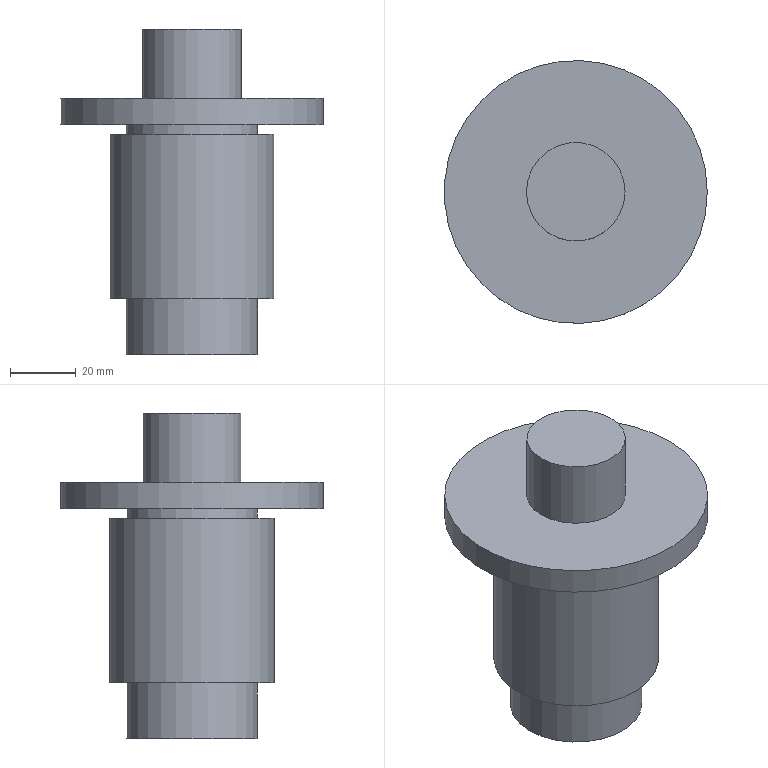Component | NX | SUPPORT_BASE | 1 solid | 11 faces | box 80 x 80 x 99 mm | volume 178364 mm3 | plane 6 | cylinder 5 | commonest cylinder face diameters 40 x2 50 x1 80 x1 30 x1
STEP:
#1=CARTESIAN_POINT('',(0.,0.,0.));
#2=DIRECTION('',(0.,0.,1.));
#3=DIRECTION('',(1.,0.,0.));
#4=AXIS2_PLACEMENT_3D('',#1,#2,#3);
#5=CARTESIAN_POINT('',(577.45,0.,4.));
#6=VERTEX_POINT('',#5);
#7=CARTESIAN_POINT('',(562.45,0.,4.));
#8=DIRECTION('',(0.,0.,1.));
#9=DIRECTION('',(1.,0.,0.));
#10=AXIS2_PLACEMENT_3D('',#7,#8,#9);
#11=CIRCLE('',#10,15.);
#12=CARTESIAN_POINT('',(562.45,0.,4.));
#13=DIRECTION('',(0.,0.,1.));
#14=DIRECTION('',(1.,0.,0.));
#15=AXIS2_PLACEMENT_3D('',#12,#13,#14);
#16=PLANE('',#15);
#17=CARTESIAN_POINT('',(0.,0.));
#18=DIRECTION('',(1.,0.));
#19=AXIS2_PLACEMENT_2D('',#17,#18);
#20=CIRCLE('',#19,15.);
#21=(GEOMETRIC_REPRESENTATION_CONTEXT(2)PARAMETRIC_REPRESENTATION_CONTEXT()REPRESENTATION_CONTEXT('',''));
#22=DEFINITIONAL_REPRESENTATION('',(#20),#21);
#23=PCURVE('',#16,#22);
#24=CARTESIAN_POINT('',(562.45,0.,4.));
#25=DIRECTION('',(0.,0.,1.));
#26=DIRECTION('',(1.,0.,0.));
#27=AXIS2_PLACEMENT_3D('',#24,#25,#26);
#28=CYLINDRICAL_SURFACE('',#27,15.);
#29=CARTESIAN_POINT('',(0.,0.));
#30=DIRECTION('',(1.,0.));
#31=VECTOR('',#30,1.);
#32=LINE('',#29,#31);
#33=(GEOMETRIC_REPRESENTATION_CONTEXT(2)PARAMETRIC_REPRESENTATION_CONTEXT()REPRESENTATION_CONTEXT('',''));
#34=DEFINITIONAL_REPRESENTATION('',(#32),#33);
#35=PCURVE('',#28,#34);
#36=SURFACE_CURVE('',#11,(#23,#35),.PCURVE_S1.);
#37=EDGE_CURVE('',#6,#6,#36,.T.);
#38=ORIENTED_EDGE('',*,*,#37,.T.);
#39=EDGE_LOOP('',(#38));
#40=FACE_BOUND('',#39,.T.);
#41=ADVANCED_FACE('',(#40),#16,.T.);
#42=CARTESIAN_POINT('',(582.45,0.,-95.));
#43=VERTEX_POINT('',#42);
#44=CARTESIAN_POINT('',(562.45,0.,-95.));
#45=DIRECTION('',(0.,0.,1.));
#46=DIRECTION('',(1.,0.,0.));
#47=AXIS2_PLACEMENT_3D('',#44,#45,#46);
#48=CIRCLE('',#47,20.);
#49=CARTESIAN_POINT('',(562.45,0.,-95.));
#50=DIRECTION('',(0.,0.,1.));
#51=DIRECTION('',(1.,0.,0.));
#52=AXIS2_PLACEMENT_3D('',#49,#50,#51);
#53=PLANE('',#52);
#54=CARTESIAN_POINT('',(0.,0.));
#55=DIRECTION('',(1.,0.));
#56=AXIS2_PLACEMENT_2D('',#54,#55);
#57=CIRCLE('',#56,20.);
#58=(GEOMETRIC_REPRESENTATION_CONTEXT(2)PARAMETRIC_REPRESENTATION_CONTEXT()REPRESENTATION_CONTEXT('',''));
#59=DEFINITIONAL_REPRESENTATION('',(#57),#58);
#60=PCURVE('',#53,#59);
#61=CARTESIAN_POINT('',(562.45,0.,4.));
#62=DIRECTION('',(0.,0.,1.));
#63=DIRECTION('',(1.,0.,0.));
#64=AXIS2_PLACEMENT_3D('',#61,#62,#63);
#65=CYLINDRICAL_SURFACE('',#64,20.);
#66=CARTESIAN_POINT('',(0.,-99.));
#67=DIRECTION('',(1.,0.));
#68=VECTOR('',#67,1.);
#69=LINE('',#66,#68);
#70=(GEOMETRIC_REPRESENTATION_CONTEXT(2)PARAMETRIC_REPRESENTATION_CONTEXT()REPRESENTATION_CONTEXT('',''));
#71=DEFINITIONAL_REPRESENTATION('',(#69),#70);
#72=PCURVE('',#65,#71);
#73=SURFACE_CURVE('',#48,(#60,#72),.PCURVE_S1.);
#74=EDGE_CURVE('',#43,#43,#73,.T.);
#75=ORIENTED_EDGE('',*,*,#74,.F.);
#76=EDGE_LOOP('',(#75));
#77=FACE_BOUND('',#76,.T.);
#78=ADVANCED_FACE('',(#77),#53,.F.);
#79=ORIENTED_EDGE('',*,*,#74,.T.);
#80=CARTESIAN_POINT('',(582.45,0.,-78.));
#81=VERTEX_POINT('',#80);
#82=CARTESIAN_POINT('',(582.45,0.,-95.));
#83=CARTESIAN_POINT('',(582.45,0.,-78.));
#84=B_SPLINE_CURVE_WITH_KNOTS('',1,(#82,#83),.UNSPECIFIED.,.F.,.F.,(2,2),(-99.,-82.),.PIECEWISE_BEZIER_KNOTS.);
#85=CARTESIAN_POINT('',(6.283,0.));
#86=DIRECTION('',(0.,1.));
#87=VECTOR('',#86,1.);
#88=LINE('',#85,#87);
#89=(GEOMETRIC_REPRESENTATION_CONTEXT(2)PARAMETRIC_REPRESENTATION_CONTEXT()REPRESENTATION_CONTEXT('',''));
#90=DEFINITIONAL_REPRESENTATION('',(#88),#89);
#91=PCURVE('',#65,#90);
#92=CARTESIAN_POINT('',(0.,0.));
#93=DIRECTION('',(0.,1.));
#94=VECTOR('',#93,1.);
#95=LINE('',#92,#94);
#96=(GEOMETRIC_REPRESENTATION_CONTEXT(2)PARAMETRIC_REPRESENTATION_CONTEXT()REPRESENTATION_CONTEXT('',''));
#97=DEFINITIONAL_REPRESENTATION('',(#95),#96);
#98=PCURVE('',#65,#97);
#99=SEAM_CURVE('',#84,(#91,#98),.PCURVE_S1.);
#100=EDGE_CURVE('',#43,#81,#99,.T.);
#101=ORIENTED_EDGE('',*,*,#100,.T.);
#102=CARTESIAN_POINT('',(562.45,0.,-78.));
#103=DIRECTION('',(0.,0.,1.));
#104=DIRECTION('',(1.,0.,0.));
#105=AXIS2_PLACEMENT_3D('',#102,#103,#104);
#106=CIRCLE('',#105,20.);
#107=CARTESIAN_POINT('',(0.,-82.));
#108=DIRECTION('',(1.,0.));
#109=VECTOR('',#108,1.);
#110=LINE('',#107,#109);
#111=(GEOMETRIC_REPRESENTATION_CONTEXT(2)PARAMETRIC_REPRESENTATION_CONTEXT()REPRESENTATION_CONTEXT('',''));
#112=DEFINITIONAL_REPRESENTATION('',(#110),#111);
#113=PCURVE('',#65,#112);
#114=CARTESIAN_POINT('',(562.45,-25.,-78.));
#115=DIRECTION('',(0.,0.,-1.));
#116=DIRECTION('',(-1.,0.,0.));
#117=AXIS2_PLACEMENT_3D('',#114,#115,#116);
#118=PLANE('',#117);
#119=CARTESIAN_POINT('',(-20.,25.));
#120=CARTESIAN_POINT('',(-20.,59.641));
#121=CARTESIAN_POINT('',(10.,42.321));
#122=CARTESIAN_POINT('',(40.,25.));
#123=CARTESIAN_POINT('',(10.,7.679));
#124=CARTESIAN_POINT('',(-20.,-9.641));
#125=CARTESIAN_POINT('',(-20.,25.));
#126=(BOUNDED_CURVE()B_SPLINE_CURVE(2,(#119,#120,#121,#122,#123,#124,#125),.UNSPECIFIED.,.T.,.F.)B_SPLINE_CURVE_WITH_KNOTS((1,2,2,2,2,1),(-2.094,0.,2.094,4.189,6.283,8.378),.UNSPECIFIED.)CURVE()GEOMETRIC_REPRESENTATION_ITEM()RATIONAL_B_SPLINE_CURVE((1.,0.5,1.,0.5,1.,0.5,1.))REPRESENTATION_ITEM(''));
#127=(GEOMETRIC_REPRESENTATION_CONTEXT(2)PARAMETRIC_REPRESENTATION_CONTEXT()REPRESENTATION_CONTEXT('',''));
#128=DEFINITIONAL_REPRESENTATION('',(#126),#127);
#129=PCURVE('',#118,#128);
#130=SURFACE_CURVE('',#106,(#113,#129),.PCURVE_S1.);
#131=EDGE_CURVE('',#81,#81,#130,.T.);
#132=ORIENTED_EDGE('',*,*,#131,.F.);
#133=ORIENTED_EDGE('',*,*,#100,.F.);
#134=EDGE_LOOP('',(#79,#101,#132,#133));
#135=FACE_BOUND('',#134,.T.);
#136=ADVANCED_FACE('',(#135),#65,.T.);
#137=ORIENTED_EDGE('',*,*,#131,.T.);
#138=EDGE_LOOP('',(#137));
#139=FACE_BOUND('',#138,.T.);
#140=CARTESIAN_POINT('',(587.45,0.,-78.));
#141=VERTEX_POINT('',#140);
#142=CARTESIAN_POINT('',(562.45,0.,-78.));
#143=DIRECTION('',(0.,0.,1.));
#144=DIRECTION('',(1.,0.,0.));
#145=AXIS2_PLACEMENT_3D('',#142,#143,#144);
#146=CIRCLE('',#145,25.);
#147=CARTESIAN_POINT('',(-25.,25.));
#148=CARTESIAN_POINT('',(-25.,68.301));
#149=CARTESIAN_POINT('',(12.5,46.651));
#150=CARTESIAN_POINT('',(50.,25.));
#151=CARTESIAN_POINT('',(12.5,3.349));
#152=CARTESIAN_POINT('',(-25.,-18.301));
#153=CARTESIAN_POINT('',(-25.,25.));
#154=(BOUNDED_CURVE()B_SPLINE_CURVE(2,(#147,#148,#149,#150,#151,#152,#153),.UNSPECIFIED.,.T.,.F.)B_SPLINE_CURVE_WITH_KNOTS((1,2,2,2,2,1),(-2.094,0.,2.094,4.189,6.283,8.378),.UNSPECIFIED.)CURVE()GEOMETRIC_REPRESENTATION_ITEM()RATIONAL_B_SPLINE_CURVE((1.,0.5,1.,0.5,1.,0.5,1.))REPRESENTATION_ITEM(''));
#155=(GEOMETRIC_REPRESENTATION_CONTEXT(2)PARAMETRIC_REPRESENTATION_CONTEXT()REPRESENTATION_CONTEXT('',''));
#156=DEFINITIONAL_REPRESENTATION('',(#154),#155);
#157=PCURVE('',#118,#156);
#158=CARTESIAN_POINT('',(562.45,0.,4.));
#159=DIRECTION('',(0.,0.,1.));
#160=DIRECTION('',(1.,0.,0.));
#161=AXIS2_PLACEMENT_3D('',#158,#159,#160);
#162=CYLINDRICAL_SURFACE('',#161,25.);
#163=CARTESIAN_POINT('',(0.,-82.));
#164=DIRECTION('',(1.,0.));
#165=VECTOR('',#164,1.);
#166=LINE('',#163,#165);
#167=(GEOMETRIC_REPRESENTATION_CONTEXT(2)PARAMETRIC_REPRESENTATION_CONTEXT()REPRESENTATION_CONTEXT('',''));
#168=DEFINITIONAL_REPRESENTATION('',(#166),#167);
#169=PCURVE('',#162,#168);
#170=SURFACE_CURVE('',#146,(#157,#169),.PCURVE_S1.);
#171=EDGE_CURVE('',#141,#141,#170,.T.);
#172=ORIENTED_EDGE('',*,*,#171,.F.);
#173=EDGE_LOOP('',(#172));
#174=FACE_BOUND('',#173,.T.);
#175=ADVANCED_FACE('',(#139,#174),#118,.T.);
#176=ORIENTED_EDGE('',*,*,#171,.T.);
#177=CARTESIAN_POINT('',(587.45,0.,-28.));
#178=VERTEX_POINT('',#177);
#179=CARTESIAN_POINT('',(587.45,0.,-78.));
#180=CARTESIAN_POINT('',(587.45,0.,-28.));
#181=B_SPLINE_CURVE_WITH_KNOTS('',1,(#179,#180),.UNSPECIFIED.,.F.,.F.,(2,2),(-82.,-32.),.PIECEWISE_BEZIER_KNOTS.);
#182=CARTESIAN_POINT('',(6.283,0.));
#183=DIRECTION('',(0.,1.));
#184=VECTOR('',#183,1.);
#185=LINE('',#182,#184);
#186=(GEOMETRIC_REPRESENTATION_CONTEXT(2)PARAMETRIC_REPRESENTATION_CONTEXT()REPRESENTATION_CONTEXT('',''));
#187=DEFINITIONAL_REPRESENTATION('',(#185),#186);
#188=PCURVE('',#162,#187);
#189=CARTESIAN_POINT('',(0.,0.));
#190=DIRECTION('',(0.,1.));
#191=VECTOR('',#190,1.);
#192=LINE('',#189,#191);
#193=(GEOMETRIC_REPRESENTATION_CONTEXT(2)PARAMETRIC_REPRESENTATION_CONTEXT()REPRESENTATION_CONTEXT('',''));
#194=DEFINITIONAL_REPRESENTATION('',(#192),#193);
#195=PCURVE('',#162,#194);
#196=SEAM_CURVE('',#181,(#188,#195),.PCURVE_S1.);
#197=EDGE_CURVE('',#141,#178,#196,.T.);
#198=ORIENTED_EDGE('',*,*,#197,.T.);
#199=CARTESIAN_POINT('',(562.45,0.,-28.));
#200=DIRECTION('',(0.,0.,1.));
#201=DIRECTION('',(1.,0.,0.));
#202=AXIS2_PLACEMENT_3D('',#199,#200,#201);
#203=CIRCLE('',#202,25.);
#204=CARTESIAN_POINT('',(0.,-32.));
#205=DIRECTION('',(1.,0.));
#206=VECTOR('',#205,1.);
#207=LINE('',#204,#206);
#208=(GEOMETRIC_REPRESENTATION_CONTEXT(2)PARAMETRIC_REPRESENTATION_CONTEXT()REPRESENTATION_CONTEXT('',''));
#209=DEFINITIONAL_REPRESENTATION('',(#207),#208);
#210=PCURVE('',#162,#209);
#211=CARTESIAN_POINT('',(562.45,-20.,-28.));
#212=DIRECTION('',(0.,0.,1.));
#213=DIRECTION('',(1.,0.,0.));
#214=AXIS2_PLACEMENT_3D('',#211,#212,#213);
#215=PLANE('',#214);
#216=CARTESIAN_POINT('',(0.,20.));
#217=DIRECTION('',(1.,0.));
#218=AXIS2_PLACEMENT_2D('',#216,#217);
#219=CIRCLE('',#218,25.);
#220=(GEOMETRIC_REPRESENTATION_CONTEXT(2)PARAMETRIC_REPRESENTATION_CONTEXT()REPRESENTATION_CONTEXT('',''));
#221=DEFINITIONAL_REPRESENTATION('',(#219),#220);
#222=PCURVE('',#215,#221);
#223=SURFACE_CURVE('',#203,(#210,#222),.PCURVE_S1.);
#224=EDGE_CURVE('',#178,#178,#223,.T.);
#225=ORIENTED_EDGE('',*,*,#224,.F.);
#226=ORIENTED_EDGE('',*,*,#197,.F.);
#227=EDGE_LOOP('',(#176,#198,#225,#226));
#228=FACE_BOUND('',#227,.T.);
#229=ADVANCED_FACE('',(#228),#162,.T.);
#230=ORIENTED_EDGE('',*,*,#224,.T.);
#231=EDGE_LOOP('',(#230));
#232=FACE_BOUND('',#231,.T.);
#233=CARTESIAN_POINT('',(582.45,0.,-28.));
#234=VERTEX_POINT('',#233);
#235=CARTESIAN_POINT('',(562.45,0.,-28.));
#236=DIRECTION('',(0.,0.,1.));
#237=DIRECTION('',(1.,0.,0.));
#238=AXIS2_PLACEMENT_3D('',#235,#236,#237);
#239=CIRCLE('',#238,20.);
#240=CARTESIAN_POINT('',(0.,20.));
#241=DIRECTION('',(1.,0.));
#242=AXIS2_PLACEMENT_2D('',#240,#241);
#243=CIRCLE('',#242,20.);
#244=(GEOMETRIC_REPRESENTATION_CONTEXT(2)PARAMETRIC_REPRESENTATION_CONTEXT()REPRESENTATION_CONTEXT('',''));
#245=DEFINITIONAL_REPRESENTATION('',(#243),#244);
#246=PCURVE('',#215,#245);
#247=CARTESIAN_POINT('',(562.45,0.,4.));
#248=DIRECTION('',(0.,0.,1.));
#249=DIRECTION('',(1.,0.,0.));
#250=AXIS2_PLACEMENT_3D('',#247,#248,#249);
#251=CYLINDRICAL_SURFACE('',#250,20.);
#252=CARTESIAN_POINT('',(0.,-32.));
#253=DIRECTION('',(1.,0.));
#254=VECTOR('',#253,1.);
#255=LINE('',#252,#254);
#256=(GEOMETRIC_REPRESENTATION_CONTEXT(2)PARAMETRIC_REPRESENTATION_CONTEXT()REPRESENTATION_CONTEXT('',''));
#257=DEFINITIONAL_REPRESENTATION('',(#255),#256);
#258=PCURVE('',#251,#257);
#259=SURFACE_CURVE('',#239,(#246,#258),.PCURVE_S1.);
#260=EDGE_CURVE('',#234,#234,#259,.T.);
#261=ORIENTED_EDGE('',*,*,#260,.F.);
#262=EDGE_LOOP('',(#261));
#263=FACE_BOUND('',#262,.T.);
#264=ADVANCED_FACE('',(#232,#263),#215,.T.);
#265=ORIENTED_EDGE('',*,*,#260,.T.);
#266=CARTESIAN_POINT('',(582.45,0.,-25.));
#267=VERTEX_POINT('',#266);
#268=CARTESIAN_POINT('',(582.45,0.,-28.));
#269=CARTESIAN_POINT('',(582.45,0.,-25.));
#270=B_SPLINE_CURVE_WITH_KNOTS('',1,(#268,#269),.UNSPECIFIED.,.F.,.F.,(2,2),(-32.,-29.),.PIECEWISE_BEZIER_KNOTS.);
#271=CARTESIAN_POINT('',(6.283,0.));
#272=DIRECTION('',(0.,1.));
#273=VECTOR('',#272,1.);
#274=LINE('',#271,#273);
#275=(GEOMETRIC_REPRESENTATION_CONTEXT(2)PARAMETRIC_REPRESENTATION_CONTEXT()REPRESENTATION_CONTEXT('',''));
#276=DEFINITIONAL_REPRESENTATION('',(#274),#275);
#277=PCURVE('',#251,#276);
#278=CARTESIAN_POINT('',(0.,0.));
#279=DIRECTION('',(0.,1.));
#280=VECTOR('',#279,1.);
#281=LINE('',#278,#280);
#282=(GEOMETRIC_REPRESENTATION_CONTEXT(2)PARAMETRIC_REPRESENTATION_CONTEXT()REPRESENTATION_CONTEXT('',''));
#283=DEFINITIONAL_REPRESENTATION('',(#281),#282);
#284=PCURVE('',#251,#283);
#285=SEAM_CURVE('',#270,(#277,#284),.PCURVE_S1.);
#286=EDGE_CURVE('',#234,#267,#285,.T.);
#287=ORIENTED_EDGE('',*,*,#286,.T.);
#288=CARTESIAN_POINT('',(562.45,0.,-25.));
#289=DIRECTION('',(0.,0.,1.));
#290=DIRECTION('',(1.,0.,0.));
#291=AXIS2_PLACEMENT_3D('',#288,#289,#290);
#292=CIRCLE('',#291,20.);
#293=CARTESIAN_POINT('',(0.,-29.));
#294=DIRECTION('',(1.,0.));
#295=VECTOR('',#294,1.);
#296=LINE('',#293,#295);
#297=(GEOMETRIC_REPRESENTATION_CONTEXT(2)PARAMETRIC_REPRESENTATION_CONTEXT()REPRESENTATION_CONTEXT('',''));
#298=DEFINITIONAL_REPRESENTATION('',(#296),#297);
#299=PCURVE('',#251,#298);
#300=CARTESIAN_POINT('',(562.45,-40.,-25.));
#301=DIRECTION('',(0.,0.,-1.));
#302=DIRECTION('',(-1.,0.,0.));
#303=AXIS2_PLACEMENT_3D('',#300,#301,#302);
#304=PLANE('',#303);
#305=CARTESIAN_POINT('',(-20.,40.));
#306=CARTESIAN_POINT('',(-20.,74.641));
#307=CARTESIAN_POINT('',(10.,57.321));
#308=CARTESIAN_POINT('',(40.,40.));
#309=CARTESIAN_POINT('',(10.,22.679));
#310=CARTESIAN_POINT('',(-20.,5.359));
#311=CARTESIAN_POINT('',(-20.,40.));
#312=(BOUNDED_CURVE()B_SPLINE_CURVE(2,(#305,#306,#307,#308,#309,#310,#311),.UNSPECIFIED.,.T.,.F.)B_SPLINE_CURVE_WITH_KNOTS((1,2,2,2,2,1),(-2.094,0.,2.094,4.189,6.283,8.378),.UNSPECIFIED.)CURVE()GEOMETRIC_REPRESENTATION_ITEM()RATIONAL_B_SPLINE_CURVE((1.,0.5,1.,0.5,1.,0.5,1.))REPRESENTATION_ITEM(''));
#313=(GEOMETRIC_REPRESENTATION_CONTEXT(2)PARAMETRIC_REPRESENTATION_CONTEXT()REPRESENTATION_CONTEXT('',''));
#314=DEFINITIONAL_REPRESENTATION('',(#312),#313);
#315=PCURVE('',#304,#314);
#316=SURFACE_CURVE('',#292,(#299,#315),.PCURVE_S1.);
#317=EDGE_CURVE('',#267,#267,#316,.T.);
#318=ORIENTED_EDGE('',*,*,#317,.F.);
#319=ORIENTED_EDGE('',*,*,#286,.F.);
#320=EDGE_LOOP('',(#265,#287,#318,#319));
#321=FACE_BOUND('',#320,.T.);
#322=ADVANCED_FACE('',(#321),#251,.T.);
#323=ORIENTED_EDGE('',*,*,#317,.T.);
#324=EDGE_LOOP('',(#323));
#325=FACE_BOUND('',#324,.T.);
#326=CARTESIAN_POINT('',(602.45,0.,-25.));
#327=VERTEX_POINT('',#326);
#328=CARTESIAN_POINT('',(562.45,0.,-25.));
#329=DIRECTION('',(0.,0.,1.));
#330=DIRECTION('',(1.,0.,0.));
#331=AXIS2_PLACEMENT_3D('',#328,#329,#330);
#332=CIRCLE('',#331,40.);
#333=CARTESIAN_POINT('',(-40.,40.));
#334=CARTESIAN_POINT('',(-40.,109.282));
#335=CARTESIAN_POINT('',(20.,74.641));
#336=CARTESIAN_POINT('',(80.,40.));
#337=CARTESIAN_POINT('',(20.,5.359));
#338=CARTESIAN_POINT('',(-40.,-29.282));
#339=CARTESIAN_POINT('',(-40.,40.));
#340=(BOUNDED_CURVE()B_SPLINE_CURVE(2,(#333,#334,#335,#336,#337,#338,#339),.UNSPECIFIED.,.T.,.F.)B_SPLINE_CURVE_WITH_KNOTS((1,2,2,2,2,1),(-2.094,0.,2.094,4.189,6.283,8.378),.UNSPECIFIED.)CURVE()GEOMETRIC_REPRESENTATION_ITEM()RATIONAL_B_SPLINE_CURVE((1.,0.5,1.,0.5,1.,0.5,1.))REPRESENTATION_ITEM(''));
#341=(GEOMETRIC_REPRESENTATION_CONTEXT(2)PARAMETRIC_REPRESENTATION_CONTEXT()REPRESENTATION_CONTEXT('',''));
#342=DEFINITIONAL_REPRESENTATION('',(#340),#341);
#343=PCURVE('',#304,#342);
#344=CARTESIAN_POINT('',(562.45,0.,4.));
#345=DIRECTION('',(0.,0.,1.));
#346=DIRECTION('',(1.,0.,0.));
#347=AXIS2_PLACEMENT_3D('',#344,#345,#346);
#348=CYLINDRICAL_SURFACE('',#347,40.);
#349=CARTESIAN_POINT('',(0.,-29.));
#350=DIRECTION('',(1.,0.));
#351=VECTOR('',#350,1.);
#352=LINE('',#349,#351);
#353=(GEOMETRIC_REPRESENTATION_CONTEXT(2)PARAMETRIC_REPRESENTATION_CONTEXT()REPRESENTATION_CONTEXT('',''));
#354=DEFINITIONAL_REPRESENTATION('',(#352),#353);
#355=PCURVE('',#348,#354);
#356=SURFACE_CURVE('',#332,(#343,#355),.PCURVE_S1.);
#357=EDGE_CURVE('',#327,#327,#356,.T.);
#358=ORIENTED_EDGE('',*,*,#357,.F.);
#359=EDGE_LOOP('',(#358));
#360=FACE_BOUND('',#359,.T.);
#361=ADVANCED_FACE('',(#325,#360),#304,.T.);
#362=ORIENTED_EDGE('',*,*,#357,.T.);
#363=CARTESIAN_POINT('',(602.45,0.,-17.));
#364=VERTEX_POINT('',#363);
#365=CARTESIAN_POINT('',(602.45,0.,-25.));
#366=CARTESIAN_POINT('',(602.45,0.,-17.));
#367=B_SPLINE_CURVE_WITH_KNOTS('',1,(#365,#366),.UNSPECIFIED.,.F.,.F.,(2,2),(-29.,-21.),.PIECEWISE_BEZIER_KNOTS.);
#368=CARTESIAN_POINT('',(6.283,0.));
#369=DIRECTION('',(0.,1.));
#370=VECTOR('',#369,1.);
#371=LINE('',#368,#370);
#372=(GEOMETRIC_REPRESENTATION_CONTEXT(2)PARAMETRIC_REPRESENTATION_CONTEXT()REPRESENTATION_CONTEXT('',''));
#373=DEFINITIONAL_REPRESENTATION('',(#371),#372);
#374=PCURVE('',#348,#373);
#375=CARTESIAN_POINT('',(0.,0.));
#376=DIRECTION('',(0.,1.));
#377=VECTOR('',#376,1.);
#378=LINE('',#375,#377);
#379=(GEOMETRIC_REPRESENTATION_CONTEXT(2)PARAMETRIC_REPRESENTATION_CONTEXT()REPRESENTATION_CONTEXT('',''));
#380=DEFINITIONAL_REPRESENTATION('',(#378),#379);
#381=PCURVE('',#348,#380);
#382=SEAM_CURVE('',#367,(#374,#381),.PCURVE_S1.);
#383=EDGE_CURVE('',#327,#364,#382,.T.);
#384=ORIENTED_EDGE('',*,*,#383,.T.);
#385=CARTESIAN_POINT('',(562.45,0.,-17.));
#386=DIRECTION('',(0.,0.,1.));
#387=DIRECTION('',(1.,0.,0.));
#388=AXIS2_PLACEMENT_3D('',#385,#386,#387);
#389=CIRCLE('',#388,40.);
#390=CARTESIAN_POINT('',(0.,-21.));
#391=DIRECTION('',(1.,0.));
#392=VECTOR('',#391,1.);
#393=LINE('',#390,#392);
#394=(GEOMETRIC_REPRESENTATION_CONTEXT(2)PARAMETRIC_REPRESENTATION_CONTEXT()REPRESENTATION_CONTEXT('',''));
#395=DEFINITIONAL_REPRESENTATION('',(#393),#394);
#396=PCURVE('',#348,#395);
#397=CARTESIAN_POINT('',(562.45,-15.,-17.));
#398=DIRECTION('',(0.,0.,1.));
#399=DIRECTION('',(1.,0.,0.));
#400=AXIS2_PLACEMENT_3D('',#397,#398,#399);
#401=PLANE('',#400);
#402=CARTESIAN_POINT('',(0.,15.));
#403=DIRECTION('',(1.,0.));
#404=AXIS2_PLACEMENT_2D('',#402,#403);
#405=CIRCLE('',#404,40.);
#406=(GEOMETRIC_REPRESENTATION_CONTEXT(2)PARAMETRIC_REPRESENTATION_CONTEXT()REPRESENTATION_CONTEXT('',''));
#407=DEFINITIONAL_REPRESENTATION('',(#405),#406);
#408=PCURVE('',#401,#407);
#409=SURFACE_CURVE('',#389,(#396,#408),.PCURVE_S1.);
#410=EDGE_CURVE('',#364,#364,#409,.T.);
#411=ORIENTED_EDGE('',*,*,#410,.F.);
#412=ORIENTED_EDGE('',*,*,#383,.F.);
#413=EDGE_LOOP('',(#362,#384,#411,#412));
#414=FACE_BOUND('',#413,.T.);
#415=ADVANCED_FACE('',(#414),#348,.T.);
#416=ORIENTED_EDGE('',*,*,#410,.T.);
#417=EDGE_LOOP('',(#416));
#418=FACE_BOUND('',#417,.T.);
#419=CARTESIAN_POINT('',(577.45,0.,-17.));
#420=VERTEX_POINT('',#419);
#421=CARTESIAN_POINT('',(562.45,0.,-17.));
#422=DIRECTION('',(0.,0.,1.));
#423=DIRECTION('',(1.,0.,0.));
#424=AXIS2_PLACEMENT_3D('',#421,#422,#423);
#425=CIRCLE('',#424,15.);
#426=CARTESIAN_POINT('',(0.,15.));
#427=DIRECTION('',(1.,0.));
#428=AXIS2_PLACEMENT_2D('',#426,#427);
#429=CIRCLE('',#428,15.);
#430=(GEOMETRIC_REPRESENTATION_CONTEXT(2)PARAMETRIC_REPRESENTATION_CONTEXT()REPRESENTATION_CONTEXT('',''));
#431=DEFINITIONAL_REPRESENTATION('',(#429),#430);
#432=PCURVE('',#401,#431);
#433=CARTESIAN_POINT('',(0.,-21.));
#434=DIRECTION('',(1.,0.));
#435=VECTOR('',#434,1.);
#436=LINE('',#433,#435);
#437=(GEOMETRIC_REPRESENTATION_CONTEXT(2)PARAMETRIC_REPRESENTATION_CONTEXT()REPRESENTATION_CONTEXT('',''));
#438=DEFINITIONAL_REPRESENTATION('',(#436),#437);
#439=PCURVE('',#28,#438);
#440=SURFACE_CURVE('',#425,(#432,#439),.PCURVE_S1.);
#441=EDGE_CURVE('',#420,#420,#440,.T.);
#442=ORIENTED_EDGE('',*,*,#441,.F.);
#443=EDGE_LOOP('',(#442));
#444=FACE_BOUND('',#443,.T.);
#445=ADVANCED_FACE('',(#418,#444),#401,.T.);
#446=ORIENTED_EDGE('',*,*,#441,.T.);
#447=CARTESIAN_POINT('',(577.45,0.,-17.));
#448=CARTESIAN_POINT('',(577.45,0.,4.));
#449=B_SPLINE_CURVE_WITH_KNOTS('',1,(#447,#448),.UNSPECIFIED.,.F.,.F.,(2,2),(-21.,0.),.PIECEWISE_BEZIER_KNOTS.);
#450=CARTESIAN_POINT('',(6.283,0.));
#451=DIRECTION('',(0.,1.));
#452=VECTOR('',#451,1.);
#453=LINE('',#450,#452);
#454=(GEOMETRIC_REPRESENTATION_CONTEXT(2)PARAMETRIC_REPRESENTATION_CONTEXT()REPRESENTATION_CONTEXT('',''));
#455=DEFINITIONAL_REPRESENTATION('',(#453),#454);
#456=PCURVE('',#28,#455);
#457=CARTESIAN_POINT('',(0.,0.));
#458=DIRECTION('',(0.,1.));
#459=VECTOR('',#458,1.);
#460=LINE('',#457,#459);
#461=(GEOMETRIC_REPRESENTATION_CONTEXT(2)PARAMETRIC_REPRESENTATION_CONTEXT()REPRESENTATION_CONTEXT('',''));
#462=DEFINITIONAL_REPRESENTATION('',(#460),#461);
#463=PCURVE('',#28,#462);
#464=SEAM_CURVE('',#449,(#456,#463),.PCURVE_S1.);
#465=EDGE_CURVE('',#420,#6,#464,.T.);
#466=ORIENTED_EDGE('',*,*,#465,.T.);
#467=ORIENTED_EDGE('',*,*,#37,.F.);
#468=ORIENTED_EDGE('',*,*,#465,.F.);
#469=EDGE_LOOP('',(#446,#466,#467,#468));
#470=FACE_BOUND('',#469,.T.);
#471=ADVANCED_FACE('',(#470),#28,.T.);
#472=CLOSED_SHELL('',(#41,#78,#136,#175,#229,#264,#322,#361,#415,#445,#471));
#473=MANIFOLD_SOLID_BREP('',#472);
#474=(LENGTH_UNIT()NAMED_UNIT(*)SI_UNIT(.MILLI.,.METRE.));
#475=UNCERTAINTY_MEASURE_WITH_UNIT(LENGTH_MEASURE(0.00001),#474,'','');
#476=(NAMED_UNIT(*)PLANE_ANGLE_UNIT()SI_UNIT($,.RADIAN.));
#477=(NAMED_UNIT(*)SI_UNIT($,.STERADIAN.)SOLID_ANGLE_UNIT());
#478=(GEOMETRIC_REPRESENTATION_CONTEXT(3)GLOBAL_UNCERTAINTY_ASSIGNED_CONTEXT((#475))GLOBAL_UNIT_ASSIGNED_CONTEXT((#474,#476,#477))REPRESENTATION_CONTEXT('',''));
#479=ADVANCED_BREP_SHAPE_REPRESENTATION('',(#4,#473),#478);